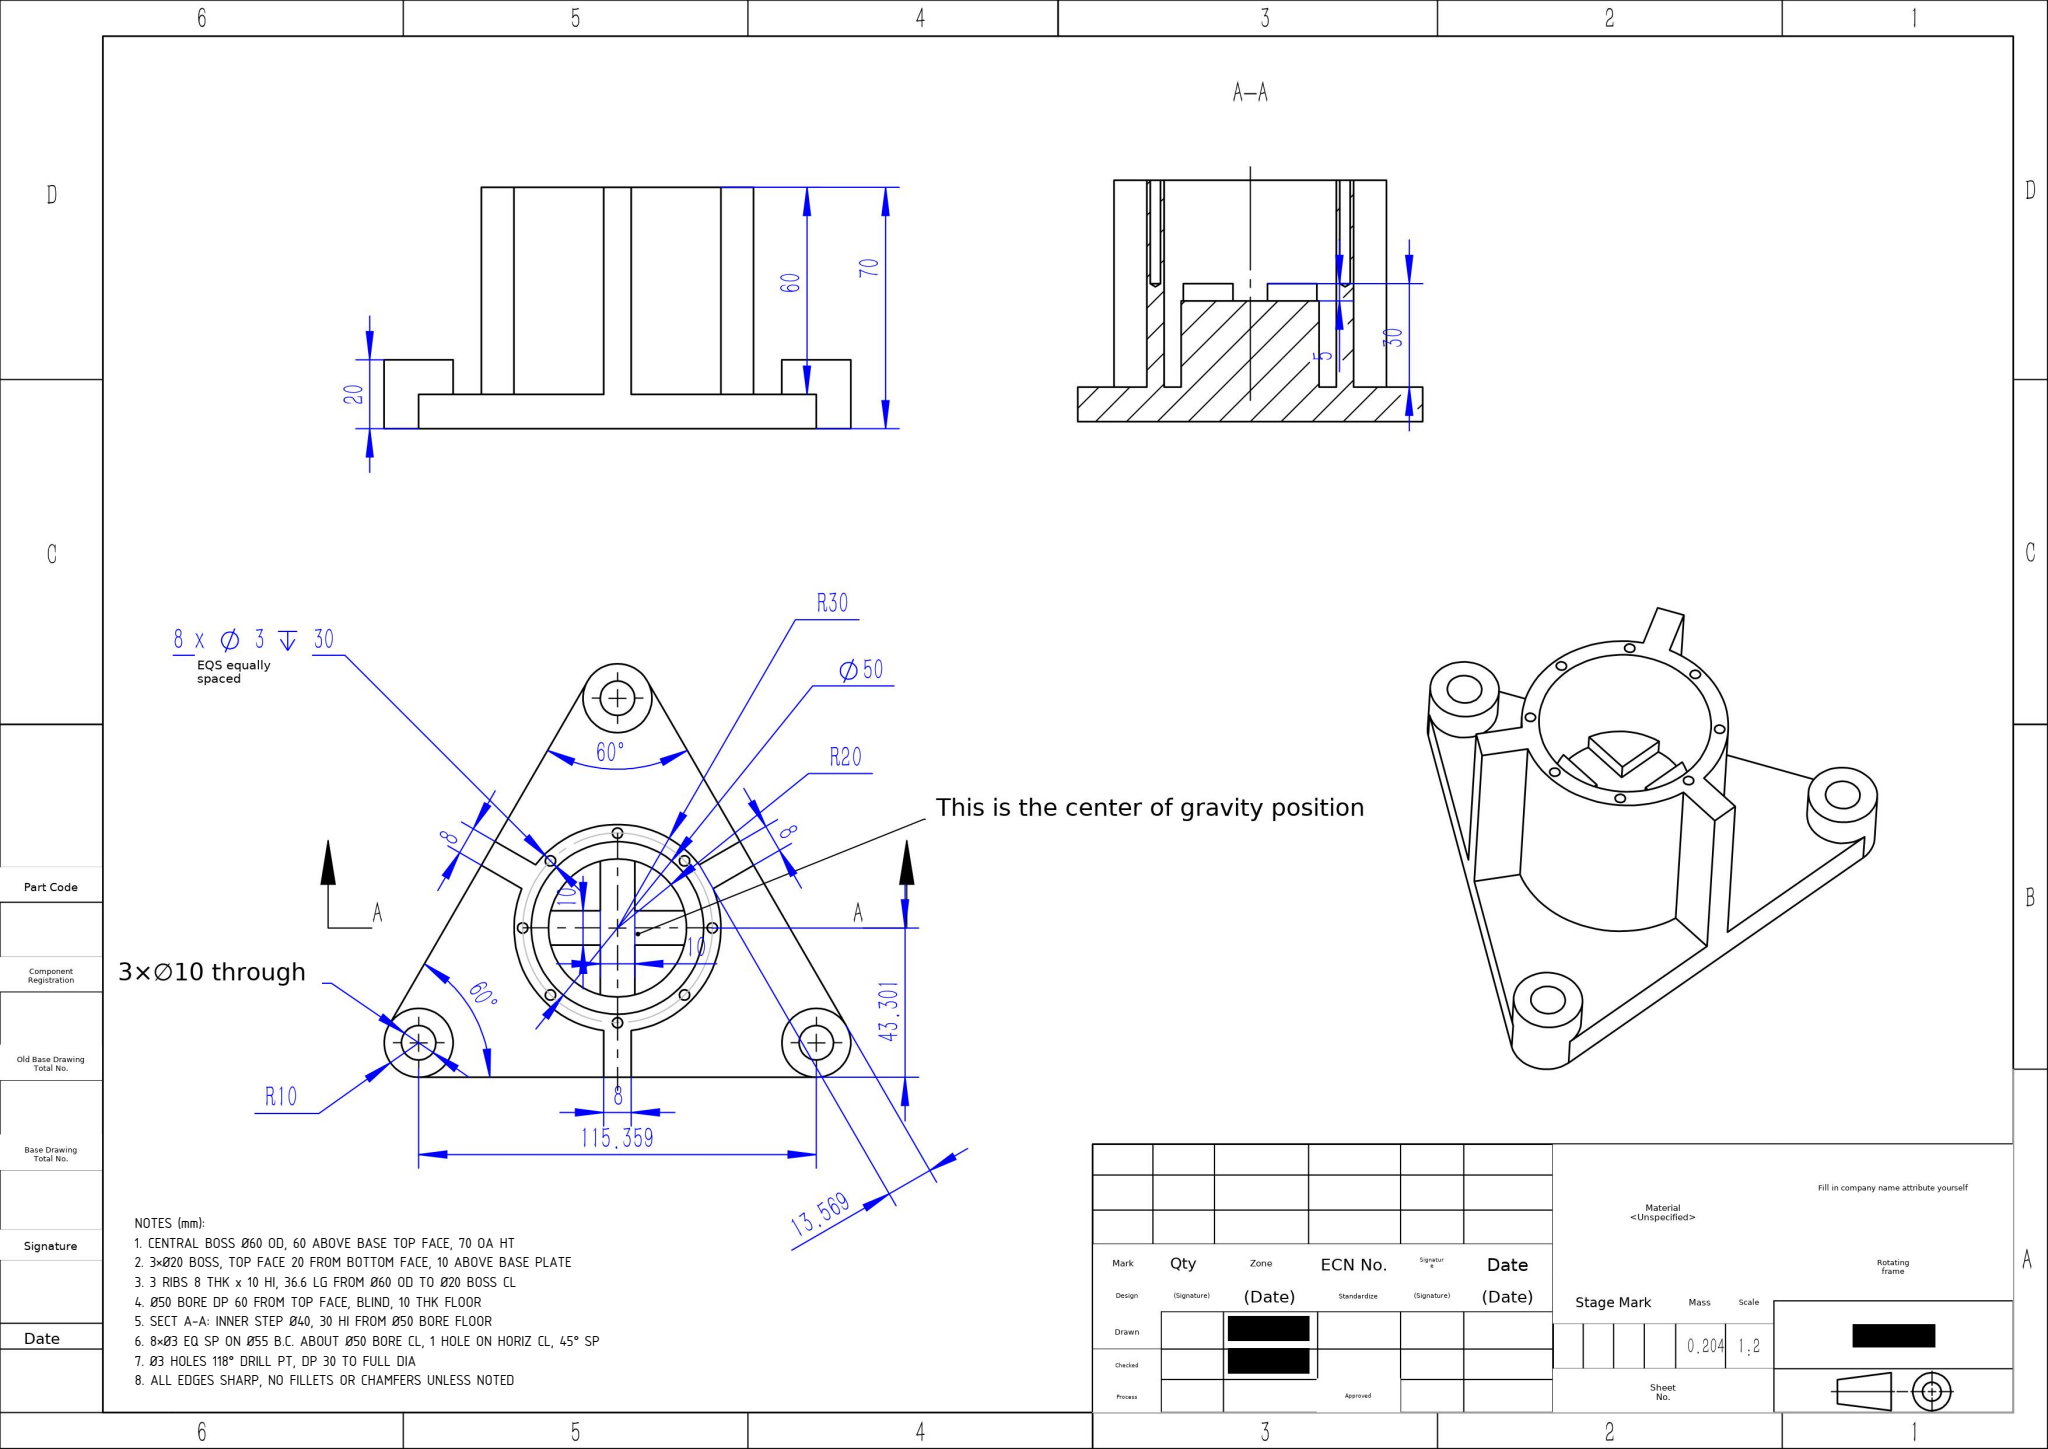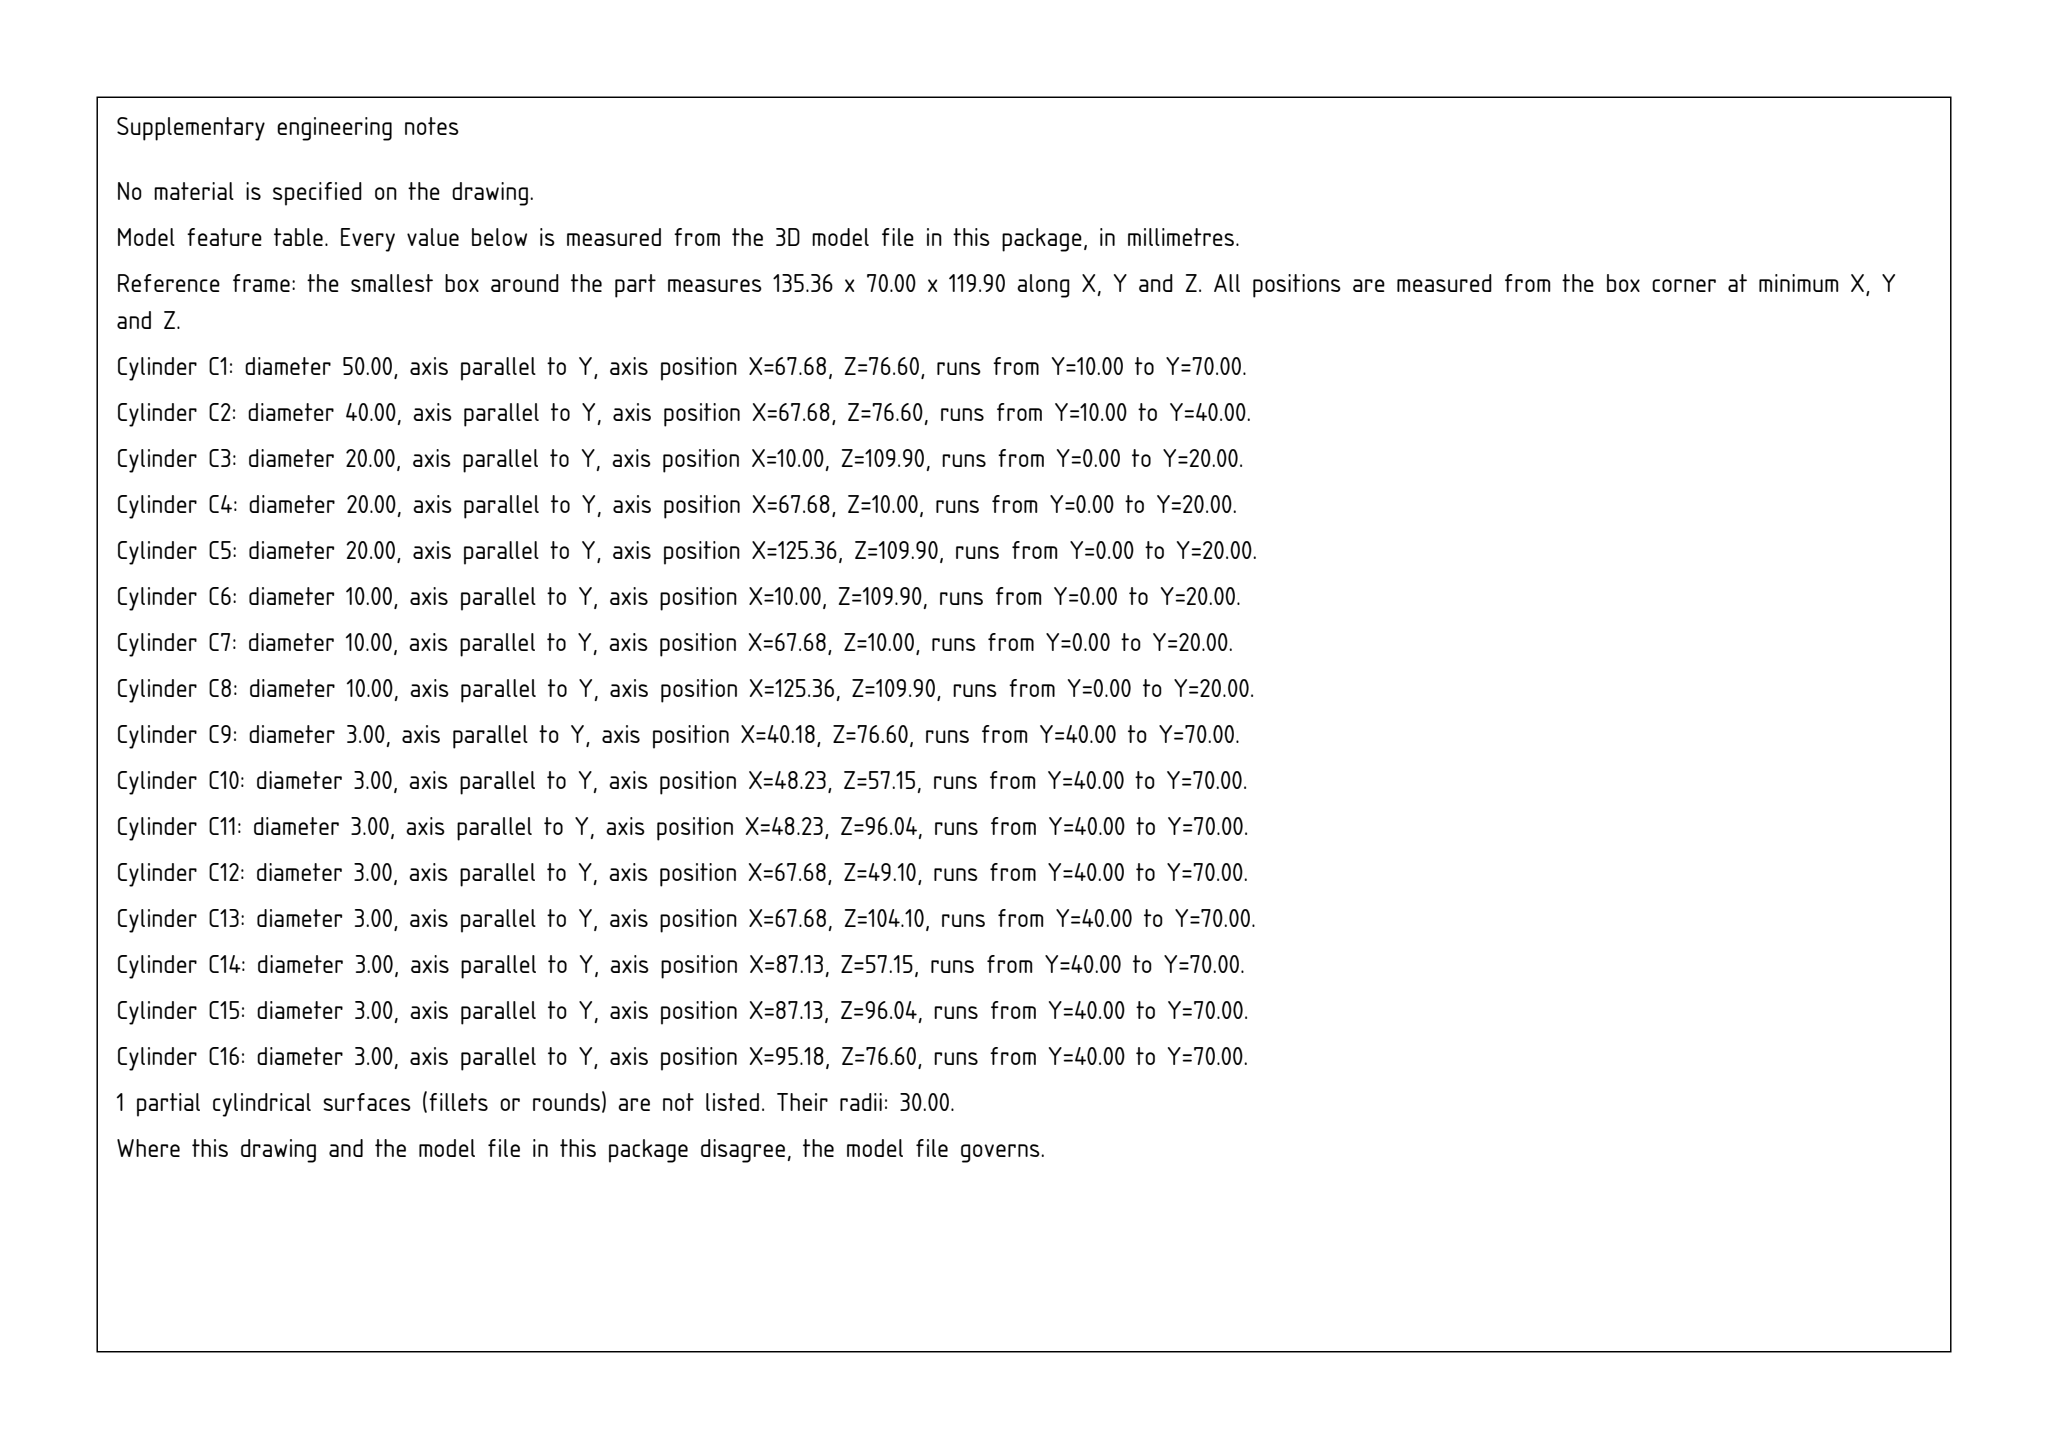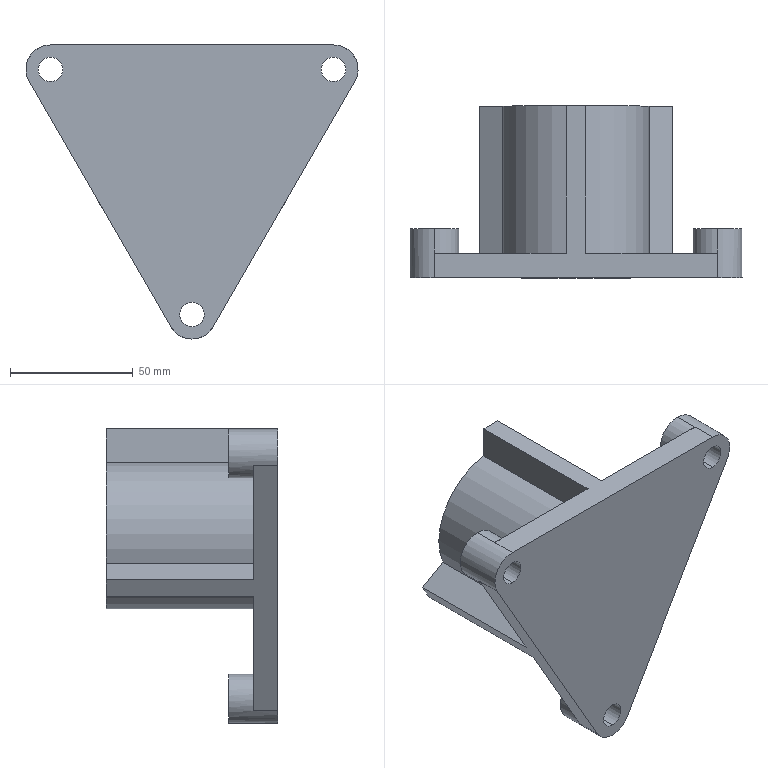Part | SolidWorks | mm | 1 solid | 83 faces | box 135.36 x 70 x 119.9 mm | volume 203732 mm3 | cylinder 36 | plane 31 | cone 16 | commonest cylinder face diameters 3 x16 10 x6 20 x6 60 x4 40 x2 50 x2
Drawing notes:
CENTRAL BOSS Ø60 OD, 60 ABOVE BASE TOP FACE, 70 OA HT | from the solid: cyl [60,y,(67.68,76.6),60]; y planes 10 (base top) and 70 (top face)
3×Ø20 BOSS, TOP FACE 20 FROM BOTTOM FACE, 10 ABOVE BASE PLATE | from the solid: cyl [20,y,...,20] and [20,y,...,10]; y planes 0,10,20
3 RIBS 8 THK x 10 HI, 36.6 LG FROM Ø60 OD TO Ø20 BOSS CL | from the solid: x planes 63.68/71.68 = 8 wide; base plate y 0-10; boss CL dist 66.6 - R30 = 36.6
Ø50 BORE DP 60 FROM TOP FACE, BLIND, 10 THK FLOOR | from the solid: cyl [50,y,(67.68,76.6),60]; top y=70, floor y=10, bottom y=0
SECT A-A: INNER STEP Ø40, 30 HI FROM Ø50 BORE FLOOR | from the solid: cyl [40,y,(67.68,76.6),30]; y planes 10, 35, 40
8×Ø3 EQ SP ON Ø55 B.C. ABOUT Ø50 BORE CL, 1 HOLE ON HORIZ CL, 45° SP | from the solid: Ø3 holes at R27.5 about boss axis (67.68,76.6) → PCD Ø55; hole at (95.18,76.6) on axis z
Ø3 HOLES 118° DRILL PT, DP 30 TO FULL DIA | from the solid: cones[118.0, ref_dia 3.0]; Ø3 cyl length 30
ALL EDGES SHARP, NO FILLETS OR CHAMFERS UNLESS NOTED | from the solid: fillet_radii: [] (no fillets in model)
build123d program:
from build123d import *

# Parameters (mm, degrees)
BOSS_EXTRUDE1_DEPTH           = 10
FILLET1_R                     = 10
SKETCH2_R                     = 25
BOSS_EXTRUDE2_DEPTH           = 60
SKETCH3_R                     = 5
CUT_EXTRUDE1_DEPTH            = 151.191
SKETCH4_R                     = 20
BOSS_EXTRUDE3_DEPTH           = 30
CUT_EXTRUDE2_DEPTH            = 5
F_3_0MM_DOWEL_PIN_HOLE1_D     = 3
F_3_0MM_DOWEL_PIN_HOLE1_DEPTH = 30
F_3_0MM_DOWEL_PIN_HOLE1_TIP   = 0.9013
BOSS_EXTRUDE4_START           = 10
SKETCH10_R                    = 10
SKETCH10_R_2                  = 5
BOSS_EXTRUDE4_DEPTH           = 10


with BuildPart() as part:
    # Sketch1 → Boss-Extrude1 (new body)
    with BuildSketch(Plane(origin=(0, 0, 0), x_dir=(1, 0, 0), z_dir=(0, 1, 0))):
        Polygon((75, 0), (-75, 0), (0, 129.904), align=None)
    extrude(amount=BOSS_EXTRUDE1_DEPTH)

    # Fillet1
    fillet1_edges = [part.edges().sort_by_distance(p)[0] for p in [
        (75, 5, 0),
        (-75, 5, 0),
        (0, 5, -129.904),
    ]]
    fillet(fillet1_edges, radius=FILLET1_R)

    # Sketch2 → Boss-Extrude2 (add)
    with BuildSketch(Plane(origin=(0, 10, 0), x_dir=(1, 0, 0), z_dir=(0, 1, 0))):
        with BuildLine():
            Line((-35.5, 68.416), (-23.749, 61.631))
            ThreePointArc((-23.749, 61.631), (0, 73.301), (23.749, 61.631))
            Line((23.749, 61.631), (35.5, 68.416))
            Line((35.5, 68.416), (39.5, 61.488))
            Line((39.5, 61.488), (27.749, 54.703))
            ThreePointArc((27.749, 54.703), (25.981, 28.301), (4, 13.569))
            Line((4, 13.569), (4, 0))
            Line((4, 0), (-4, 0))
            Line((-4, 0), (-4, 13.569))
            ThreePointArc((-4, 13.569), (-25.981, 28.301), (-27.749, 54.703))
            Line((-27.749, 54.703), (-39.5, 61.488))
            Line((-39.5, 61.488), (-35.5, 68.416))
        make_face()
        with Locations(Location((0, 43.301, 0), (0, 0, 270))):
            Circle(SKETCH2_R, mode=Mode.SUBTRACT)
    extrude(amount=BOSS_EXTRUDE2_DEPTH)

    # Sketch3 → Cut-Extrude1 (cut, through all)
    with BuildSketch(Plane(origin=(0, 10, 0), x_dir=(1, 0, 0), z_dir=(0, 1, 0))):
        with Locations(Location((-57.679, 10, 0), (0, 0, 270))):
            Circle(SKETCH3_R)
        with Locations(Location((57.679, 10, 0), (0, 0, 270))):
            Circle(SKETCH3_R)
        with Locations(Location((0, 109.904, 0), (0, 0, 270))):
            Circle(SKETCH3_R)
    extrude(amount=-CUT_EXTRUDE1_DEPTH, mode=Mode.SUBTRACT)

    # Sketch4 → Boss-Extrude3 (add)
    with BuildSketch(Plane(origin=(0, 10, 0), x_dir=(1, 0, 0), z_dir=(0, 1, 0))):
        with Locations(Location((0, 43.301, 0), (0, 0, 90))):
            Circle(SKETCH4_R)
    extrude(amount=BOSS_EXTRUDE3_DEPTH)

    # Sketch5 → Cut-Extrude2 (cut)
    with BuildSketch(Plane(origin=(0, 40, 0), x_dir=(1, 0, 0), z_dir=(0, 1, 0))):
        Polygon((-5, 64.724), (5, 64.724), (5, 48.301), (21.754, 48.301), (21.754, 38.301), (5, 38.301), (5, 21.772), (-5, 21.772), (-5, 38.301), (-21.682, 38.301), (-21.682, 48.301), (-5, 48.301), align=None)
    extrude(amount=-CUT_EXTRUDE2_DEPTH, mode=Mode.SUBTRACT)

    # 3.0mm Dowel Pin Hole1
    with Locations(Plane(origin=(0, 70, 0), x_dir=(1, 0, 0), z_dir=(0, 1, 0))):
        with Locations((-19.445, 62.747), (0, 70.801), (19.445, 62.747), (27.5, 43.301), (19.445, 23.856), (0, 15.801), (-19.445, 23.856), (-27.5, 43.301)):
            Hole(F_3_0MM_DOWEL_PIN_HOLE1_D / 2, depth=F_3_0MM_DOWEL_PIN_HOLE1_DEPTH)
            with Locations((0, 0, -(F_3_0MM_DOWEL_PIN_HOLE1_DEPTH + F_3_0MM_DOWEL_PIN_HOLE1_TIP / 2))):  # 118° drill point
                Cone(0, F_3_0MM_DOWEL_PIN_HOLE1_D / 2, F_3_0MM_DOWEL_PIN_HOLE1_TIP, mode=Mode.SUBTRACT)

    # Sketch10 → Boss-Extrude4 (add)
    # profile 1 of 3: a face of its own
    with BuildSketch(Plane(origin=(0, 10, 0), x_dir=(1, 0, 0), z_dir=(0, 1, 0)).offset(BOSS_EXTRUDE4_START)):
        with Locations(Location((-57.679, 10, 0), (0, 0, 270))):
            Circle(SKETCH10_R)
        with Locations(Location((-57.679, 10, 0), (0, 0, 270))):
            Circle(SKETCH10_R_2, mode=Mode.SUBTRACT)
    # profile 2 of 3: a face of its own
    with BuildSketch(Plane(origin=(0, 10, 0), x_dir=(1, 0, 0), z_dir=(0, 1, 0)).offset(BOSS_EXTRUDE4_START)):
        with Locations(Location((0, 109.904, 0), (0, 0, 30))):
            Circle(SKETCH10_R)
        with Locations(Location((0, 109.904, 0), (0, 0, 270))):
            Circle(SKETCH10_R_2, mode=Mode.SUBTRACT)
    # profile 3 of 3: a face of its own
    with BuildSketch(Plane(origin=(0, 10, 0), x_dir=(1, 0, 0), z_dir=(0, 1, 0)).offset(BOSS_EXTRUDE4_START)):
        with Locations(Location((57.679, 10, 0), (0, 0, 270))):
            Circle(SKETCH10_R)
        with Locations(Location((57.679, 10, 0), (0, 0, 270))):
            Circle(SKETCH10_R_2, mode=Mode.SUBTRACT)
    extrude(amount=-BOSS_EXTRUDE4_DEPTH)


solid = part.part